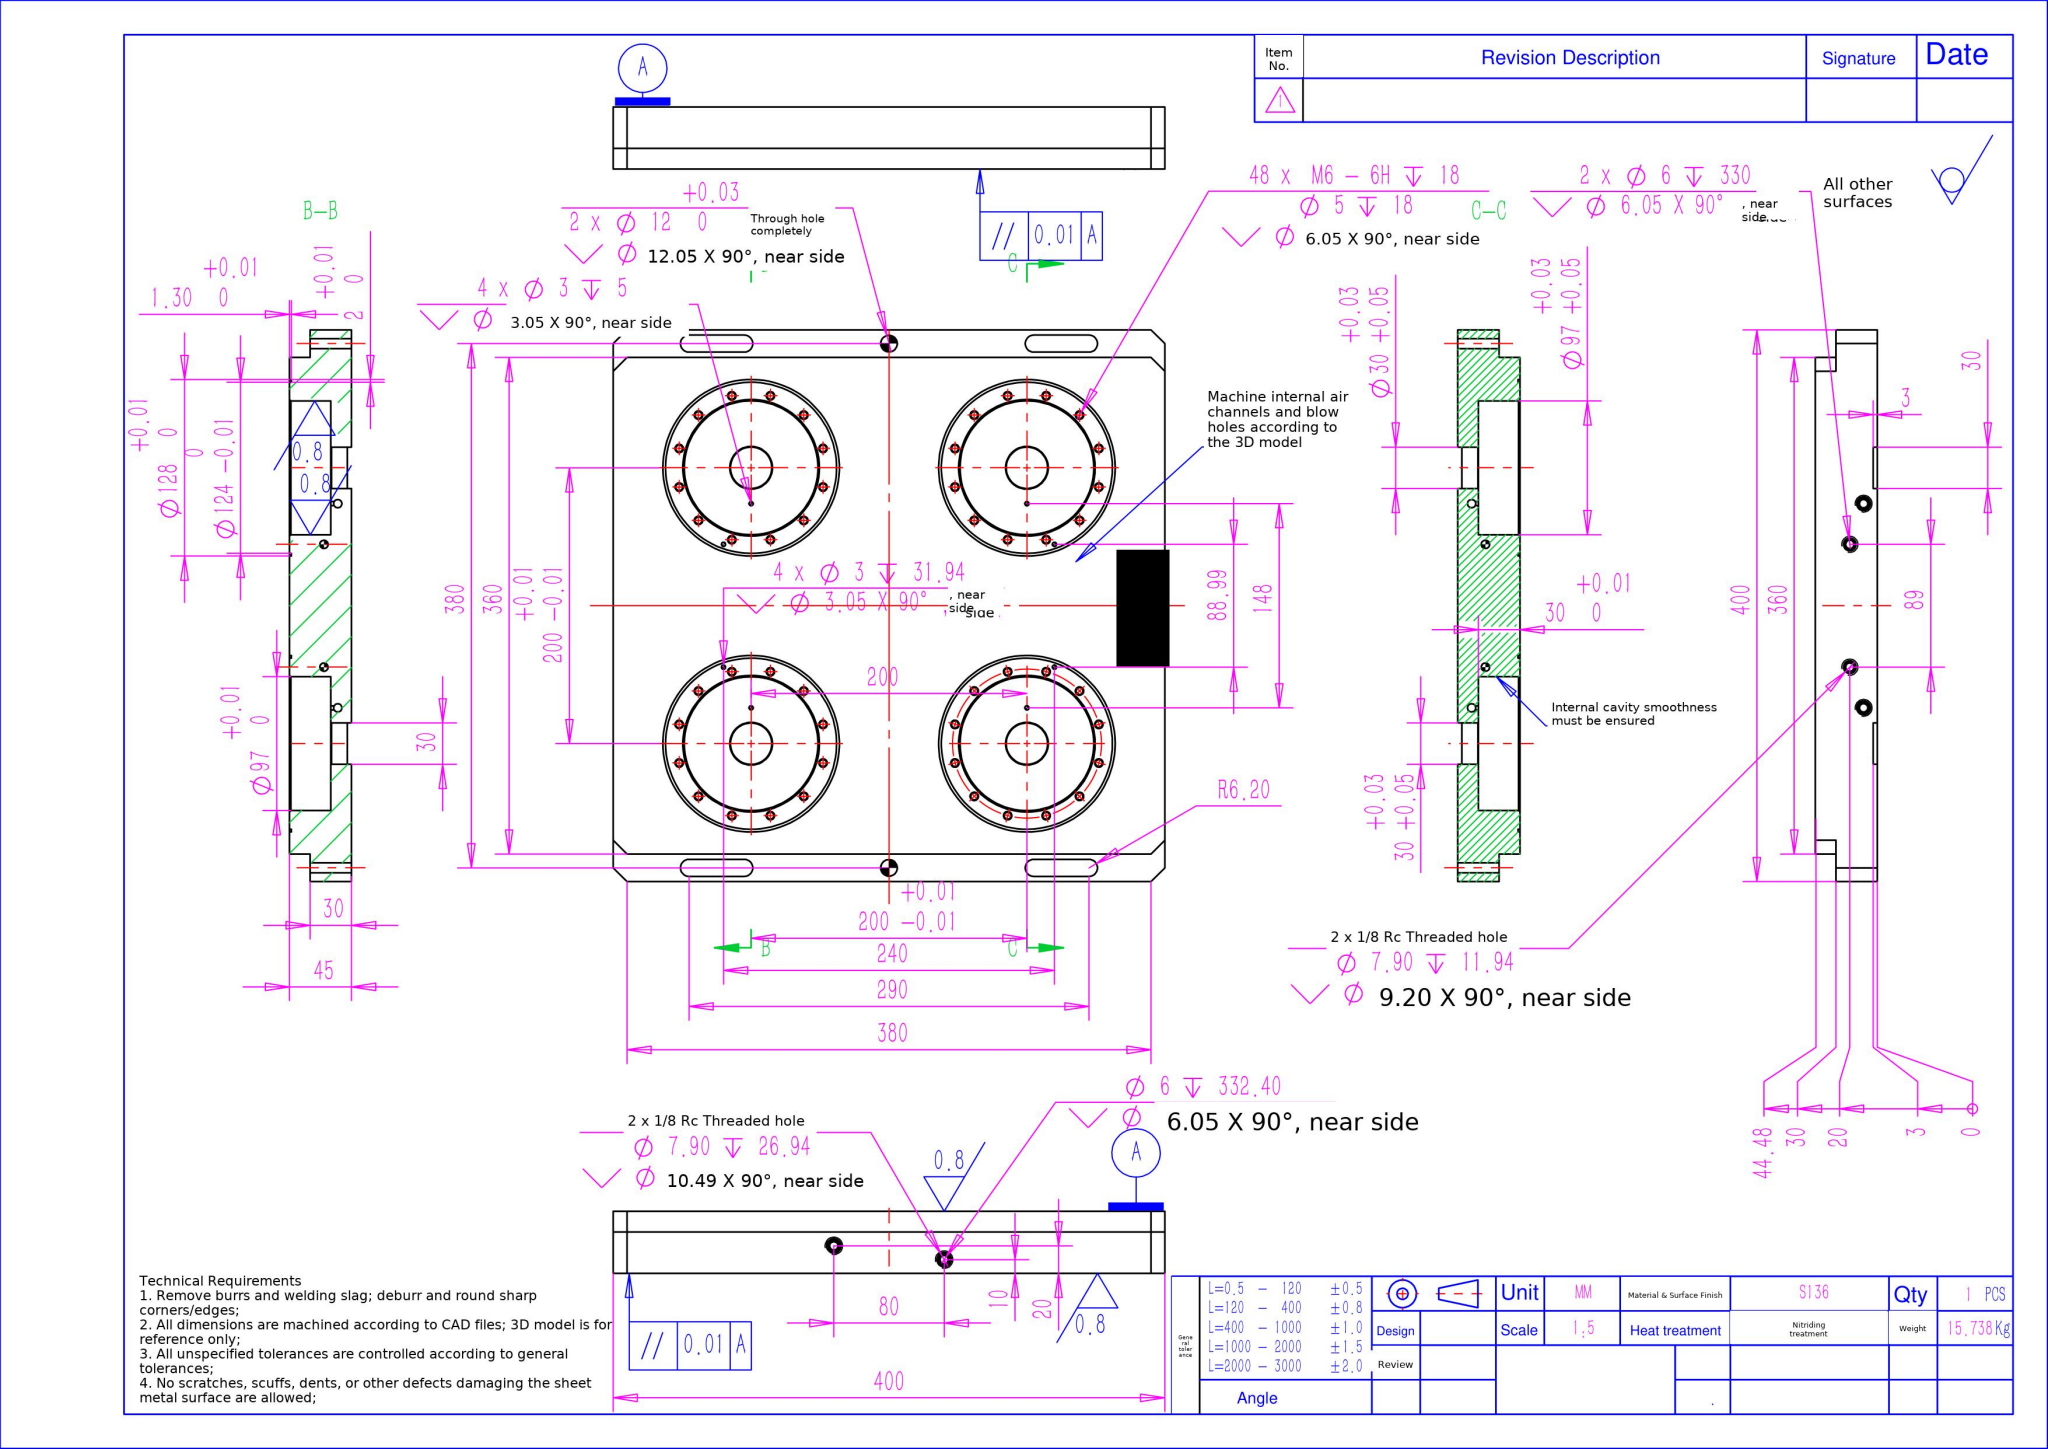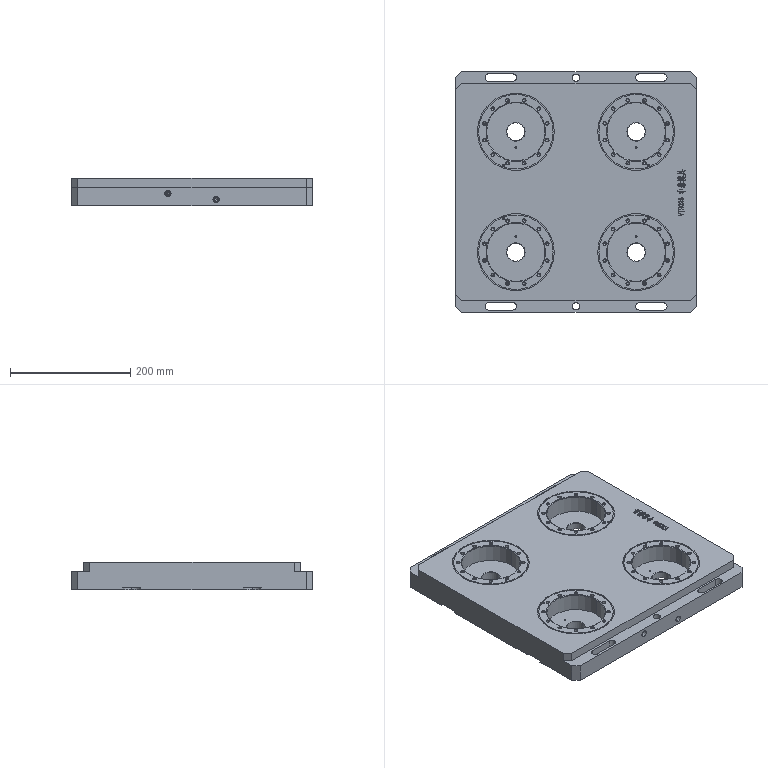Part | SolidWorks | mm | material S136 | 1 solid | 1039 faces | box 400 x 400 x 45 mm | volume 5829071 mm3 | plane 382 | cone 284 | cylinder 208 | spline 165 | commonest cylinder face diameters 5 x96 6 x28 3 x24 7.9 x12 12.4 x12 97 x8 128 x8 124 x8